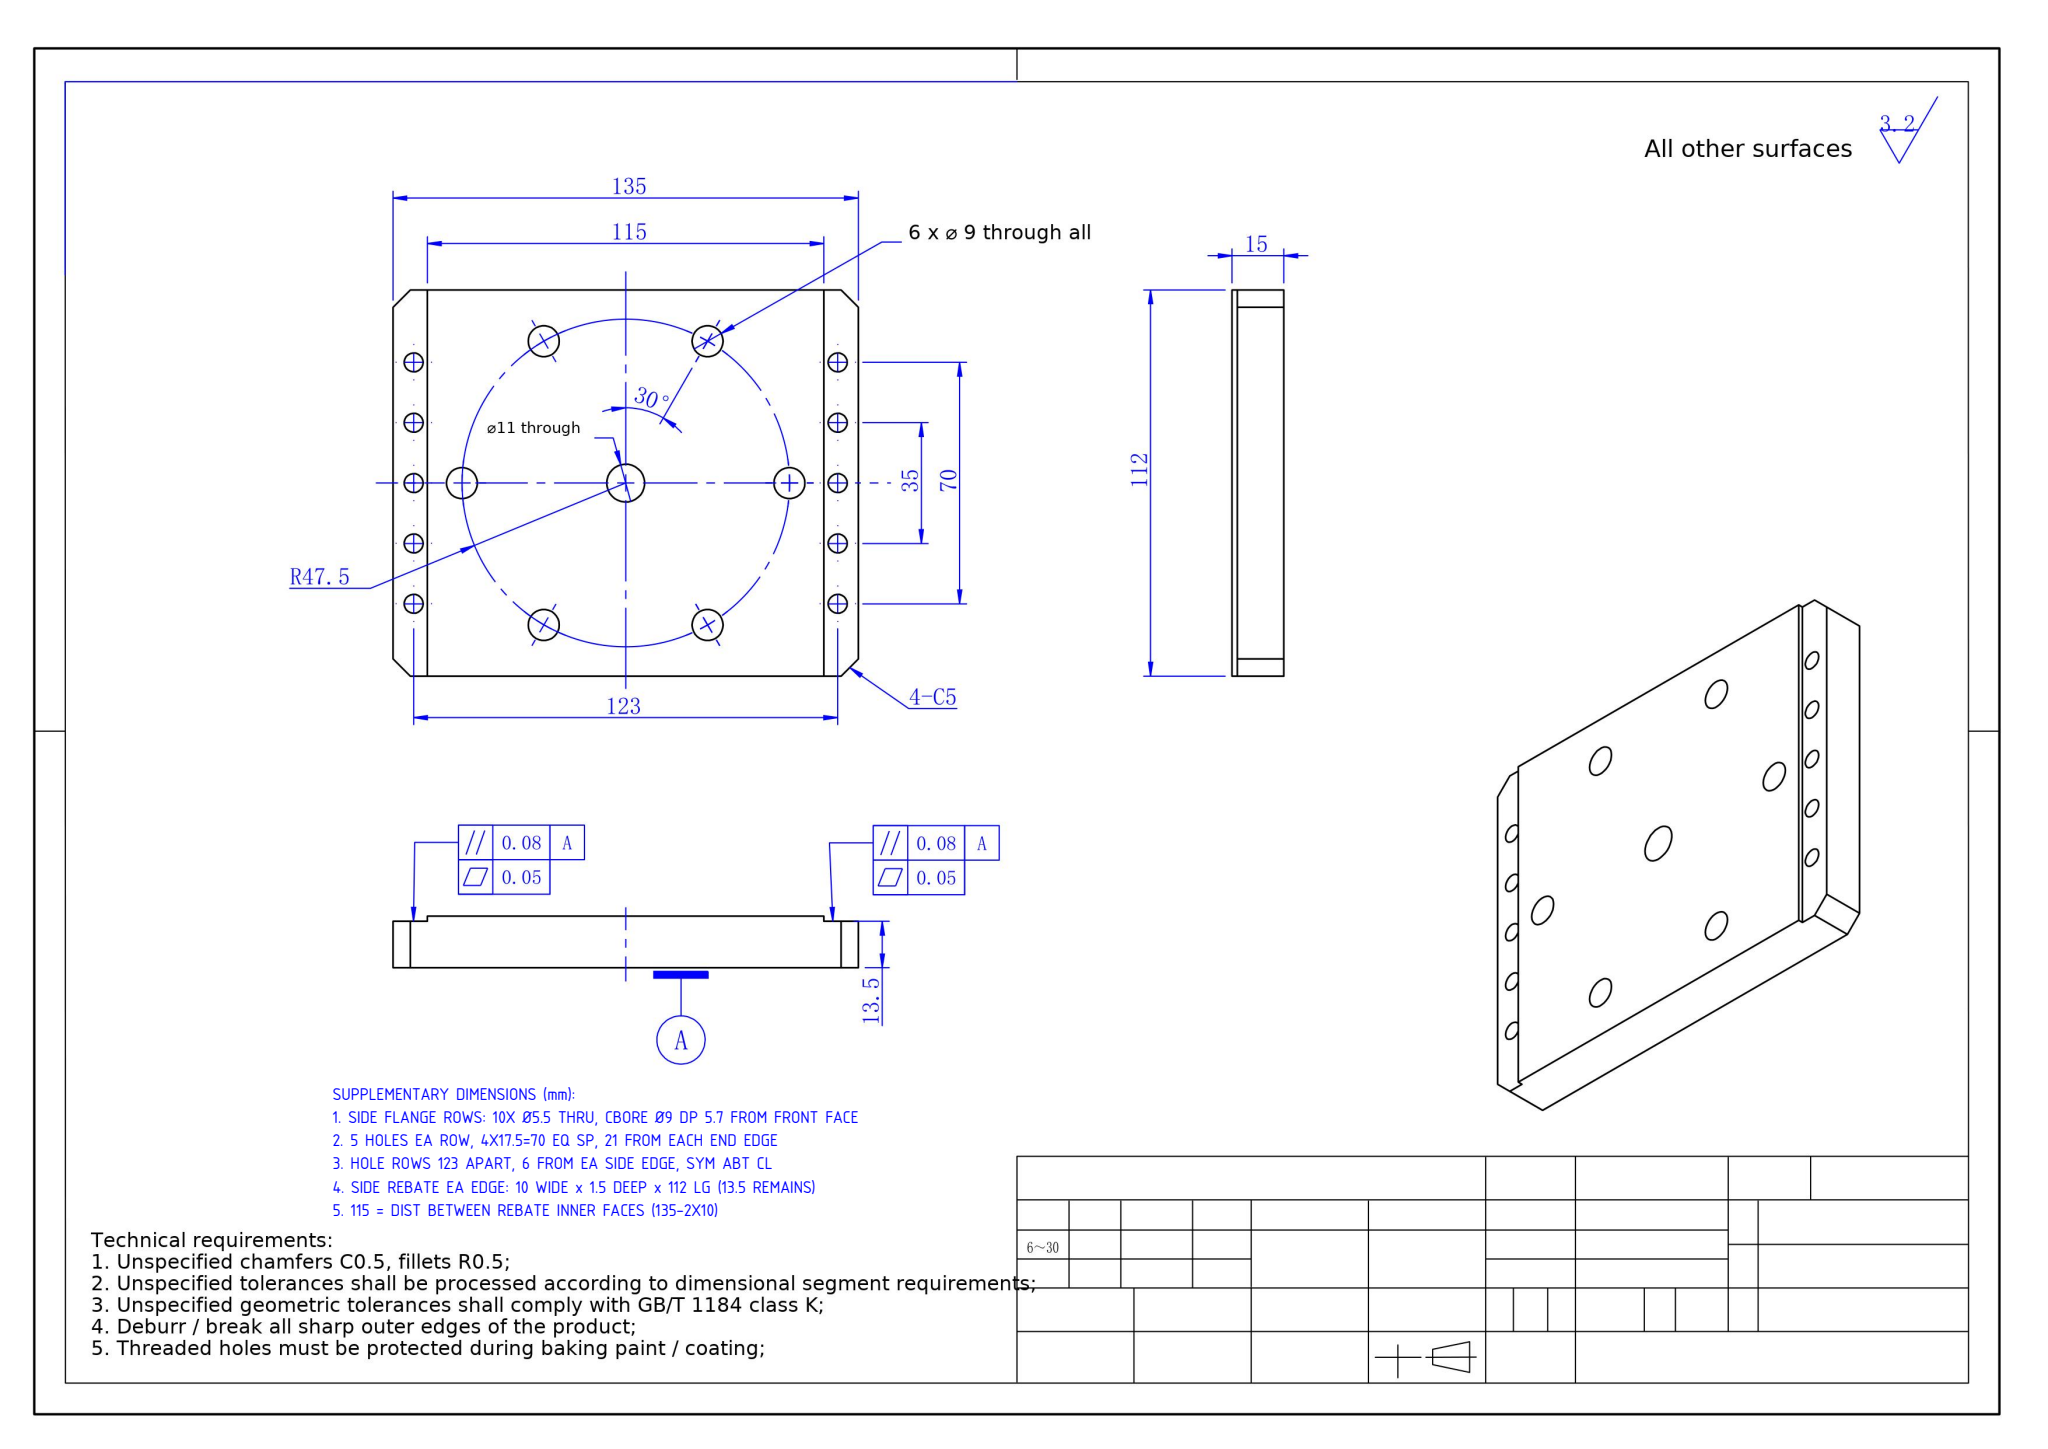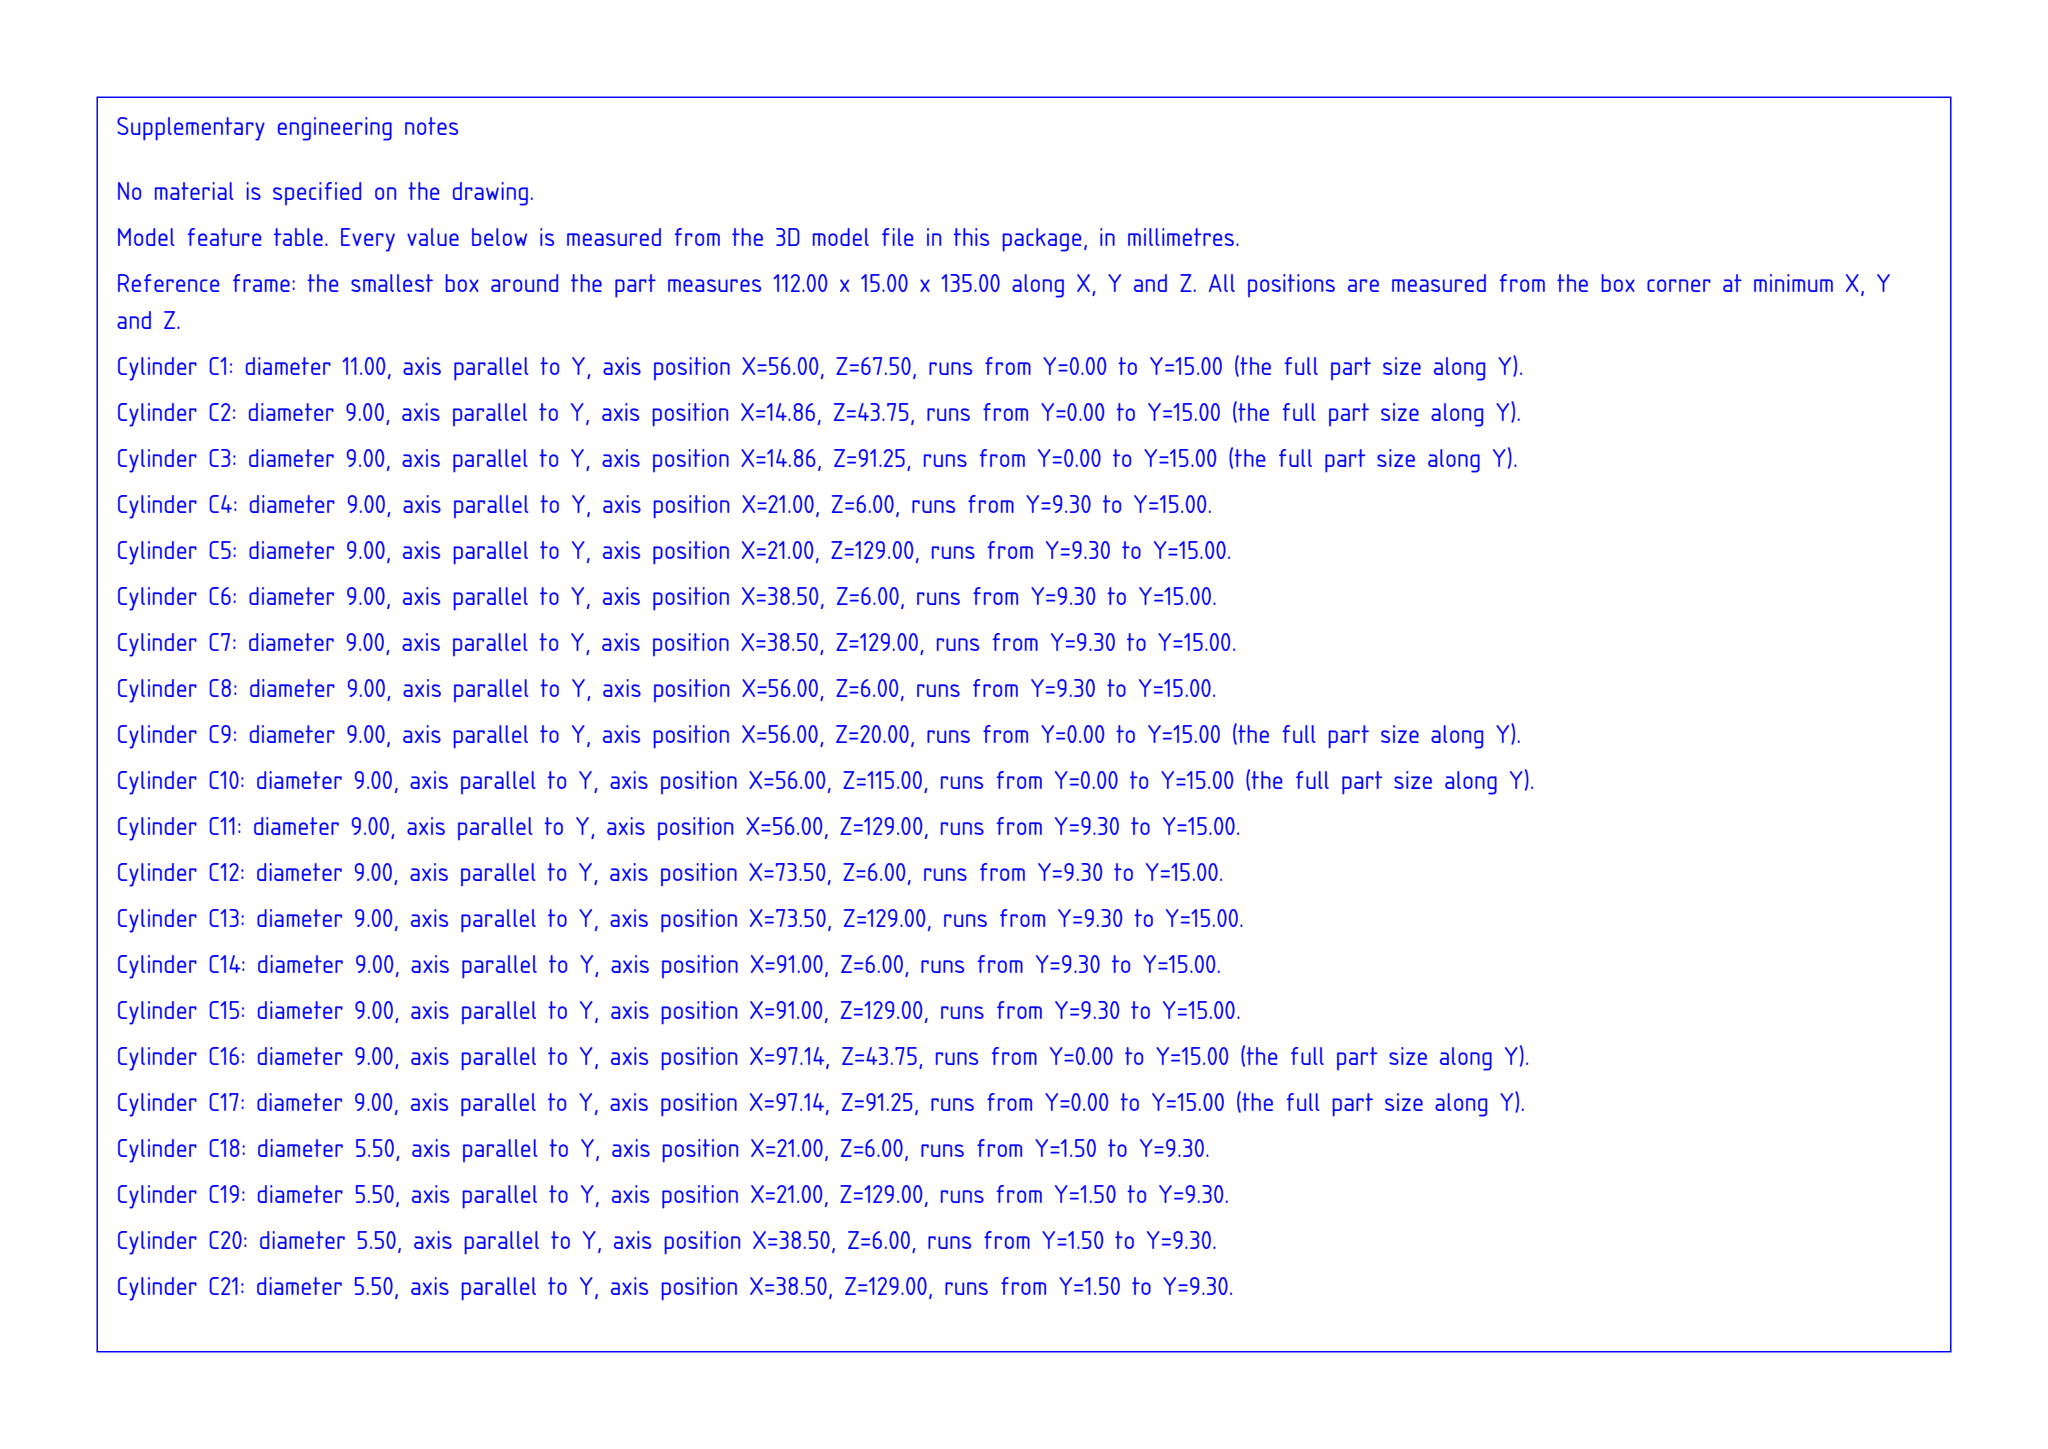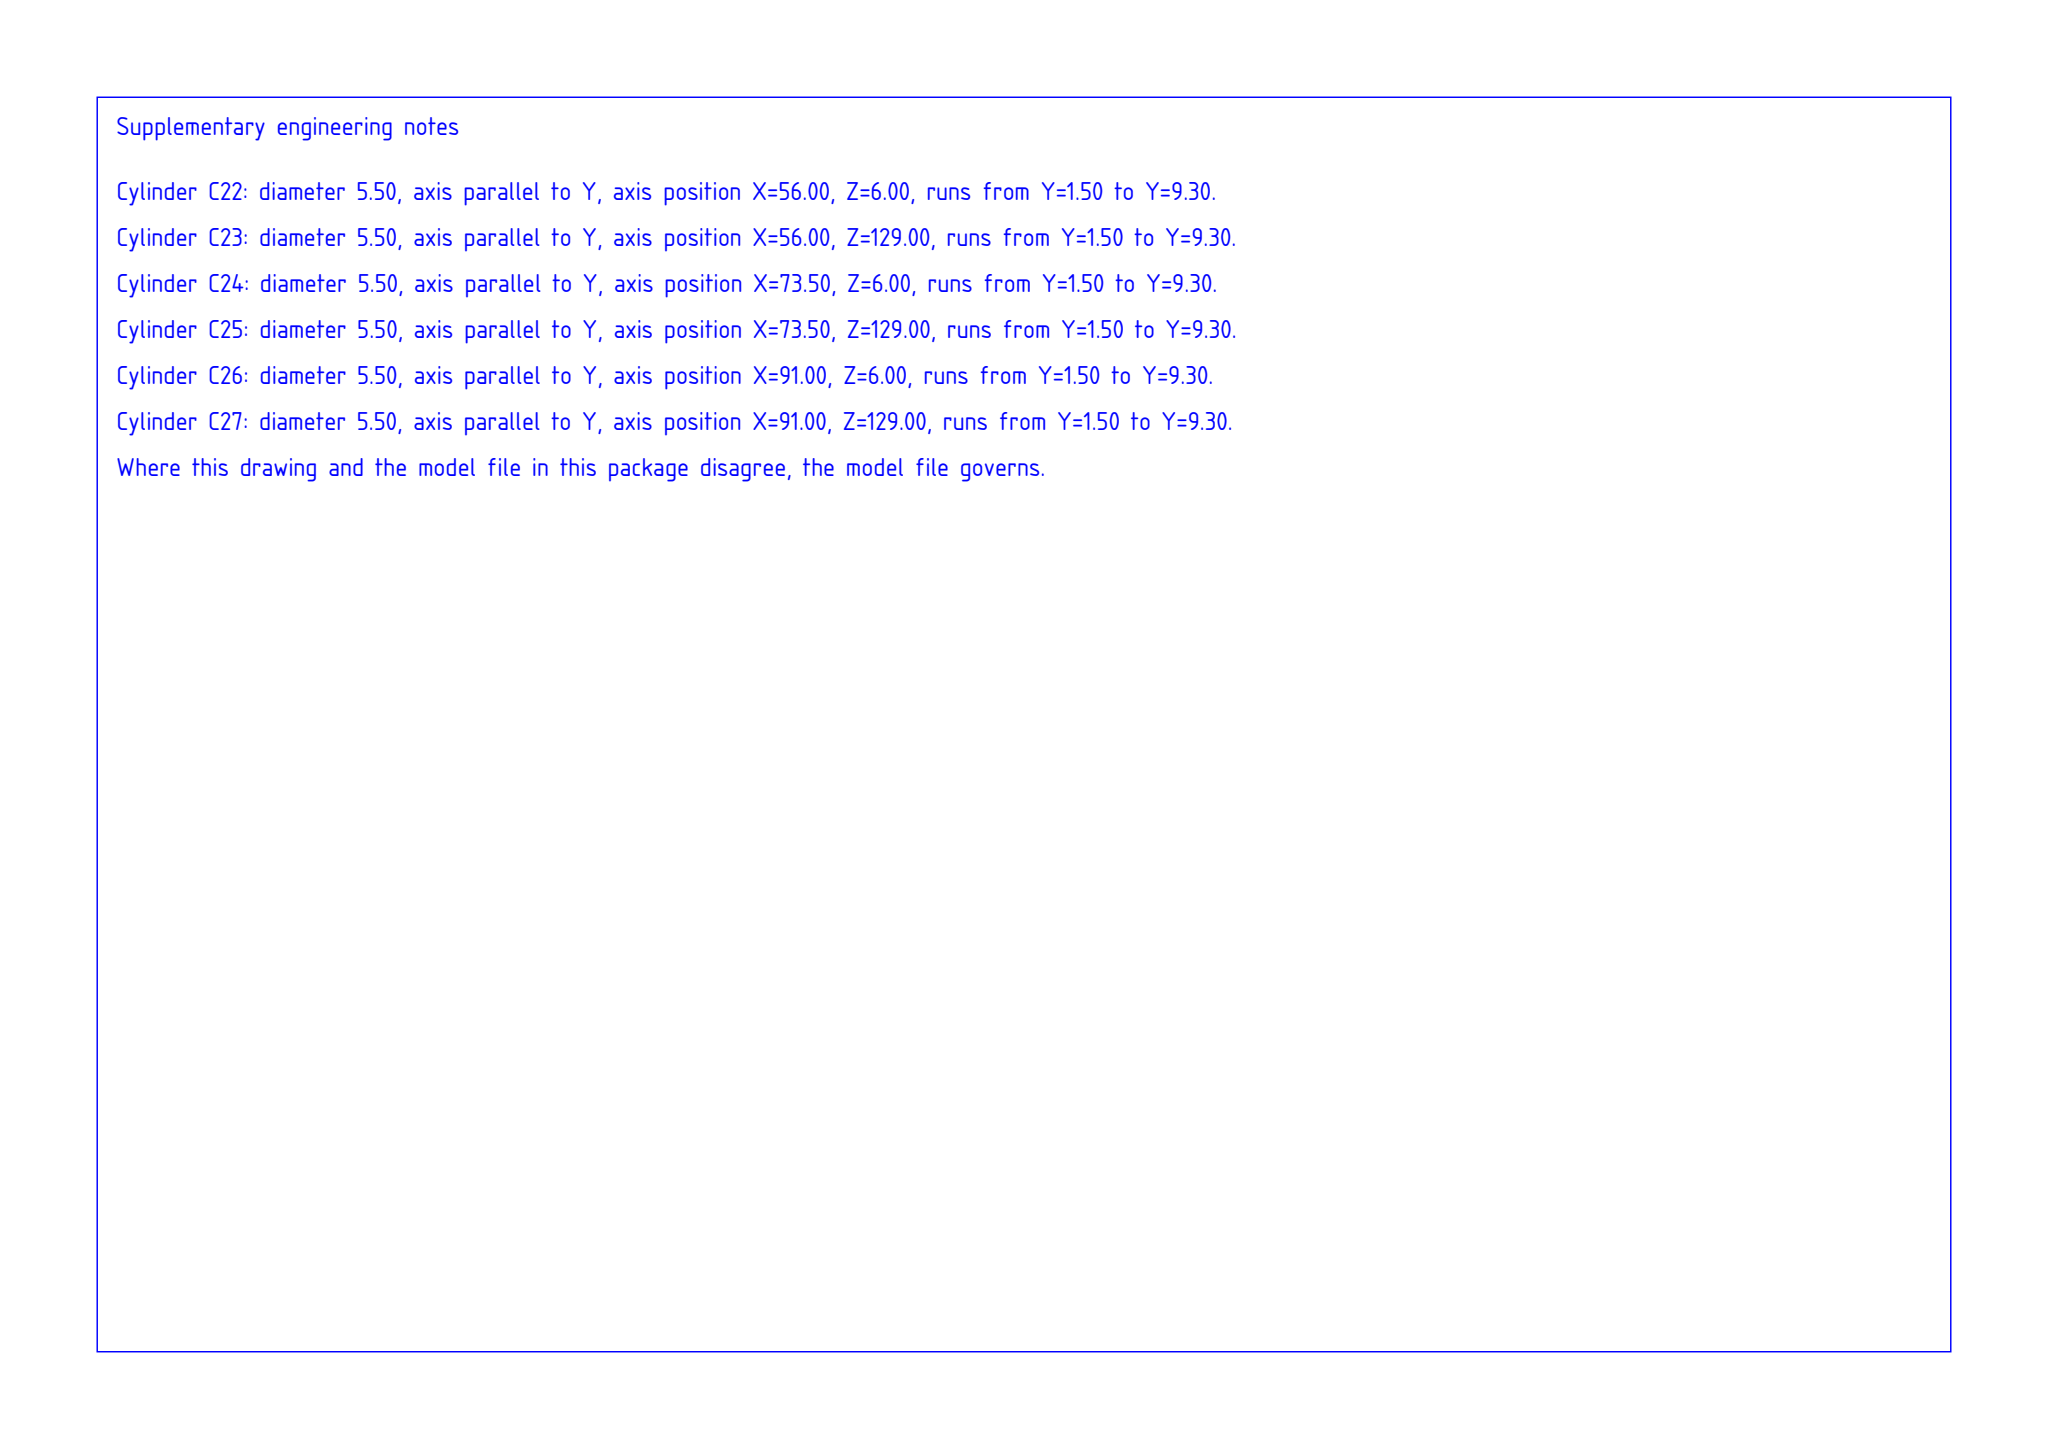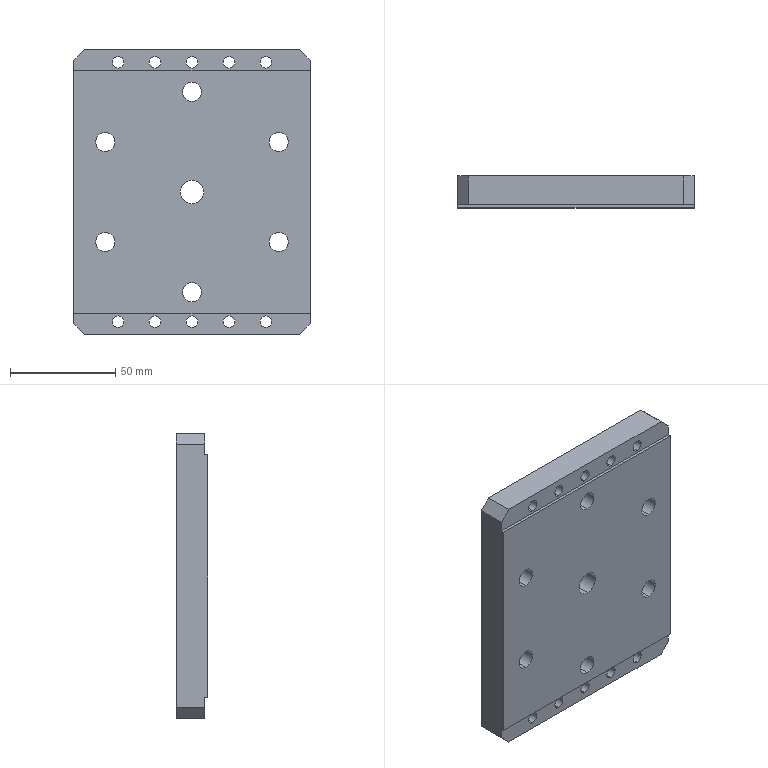Part | SolidWorks | mm | 1 solid | 78 faces | box 112 x 15 x 135 mm | volume 210135 mm3 | cylinder 54 | plane 24 | commonest cylinder face diameters 9 x32 5.5 x20 11 x2
build123d program:
from build123d import *

# Parameters (mm, degrees)
SKETCH1_W                                            = 112
SKETCH1_H                                            = 135
BOSS_EXTRUDE1_DEPTH                                  = 7.5
SKETCH3_W                                            = 112
SKETCH3_H                                            = 10
CUT_EXTRUDE1_DEPTH                                   = 1.5
CHAMFER2_SIZE                                        = 5
SKETCH4_R                                            = 5.5
CUT_EXTRUDE2_DEPTH                                   = 89.979
HOLE_SIZE_ACCORDING_TO_TYPE_OF_HEX_SOCKE_D           = 5.5
HOLE_SIZE_ACCORDING_TO_TYPE_OF_HEX_SOCKE_CBORE_D     = 9
HOLE_SIZE_ACCORDING_TO_TYPE_OF_HEX_SOCKE_CBORE_DEPTH = 5.7
M8_CLEARANCE_HOLE1_D                                 = 9
CIRPATTERN1_COUNT                                    = 6


with BuildPart() as part:
    # Sketch1 → Boss-Extrude1 (new, symmetric)
    with BuildSketch(Plane(origin=(0, 0, 0), x_dir=(1, 0, 0), z_dir=(0, 1, 0))):
        Rectangle(SKETCH1_W, SKETCH1_H)
    extrude(amount=BOSS_EXTRUDE1_DEPTH, both=True)

    # Sketch3 → Cut-Extrude1 (cut)
    with BuildSketch(Plane.XZ.offset(7.5)):
        with Locations((0, 62.5)):
            Rectangle(SKETCH3_W, SKETCH3_H)
    cut_extrude1 = extrude(amount=-CUT_EXTRUDE1_DEPTH, mode=Mode.SUBTRACT)

    # Mirror1: Cut-Extrude1 across plane
    add(cut_extrude1.mirror(Plane.XY), mode=Mode.SUBTRACT)

    # Chamfer2
    chamfer2_edges = [part.edges().sort_by_distance(p)[0] for p in [
        (56, 0.75, 67.5),
        (-56, 0.75, 67.5),
        (-56, 0.75, -67.5),
        (56, 0.75, -67.5),
    ]]
    chamfer(chamfer2_edges, length=CHAMFER2_SIZE)

    # Sketch4 → Cut-Extrude2 (cut, through all)
    with BuildSketch(Plane(origin=(0, 7.5, 0), x_dir=(1, 0, 0), z_dir=(0, 1, 0))):
        with Locations(Location((0, 0, 0), (0, 0, 270))):
            Circle(SKETCH4_R)
    extrude(amount=-CUT_EXTRUDE2_DEPTH, mode=Mode.SUBTRACT)

    # Hole Size_according to_type of hex socke (through all)
    with Locations(Plane(origin=(0, 7.5, 0), x_dir=(1, 0, 0), z_dir=(0, 1, 0))):
        with Locations((35, 61.5), (-35, 61.5), (-17.5, 61.5), (17.5, 61.5), (17.5, -61.5), (-17.5, -61.5), (-35, -61.5), (35, -61.5), (0, 61.5), (0, -61.5)):
            CounterBoreHole(HOLE_SIZE_ACCORDING_TO_TYPE_OF_HEX_SOCKE_D / 2, HOLE_SIZE_ACCORDING_TO_TYPE_OF_HEX_SOCKE_CBORE_D / 2, HOLE_SIZE_ACCORDING_TO_TYPE_OF_HEX_SOCKE_CBORE_DEPTH)

    # M8 Clearance Hole1 (through all)
    with Locations(Plane(origin=(0, 7.5, 0), x_dir=(1, 0, 0), z_dir=(0, 1, 0))):
        with Locations((0, 47.5)):
            m8_clearance_hole1 = Hole(M8_CLEARANCE_HOLE1_D / 2)

    # CirPattern1: M8 Clearance Hole1 ×6 about axis
    cirpattern1_axis = Axis((0, 0, 0), (0, 1, 0))
    for i in range(1, CIRPATTERN1_COUNT):
        add(m8_clearance_hole1.rotate(cirpattern1_axis, i * 360 / CIRPATTERN1_COUNT), mode=Mode.SUBTRACT)


solid = part.part